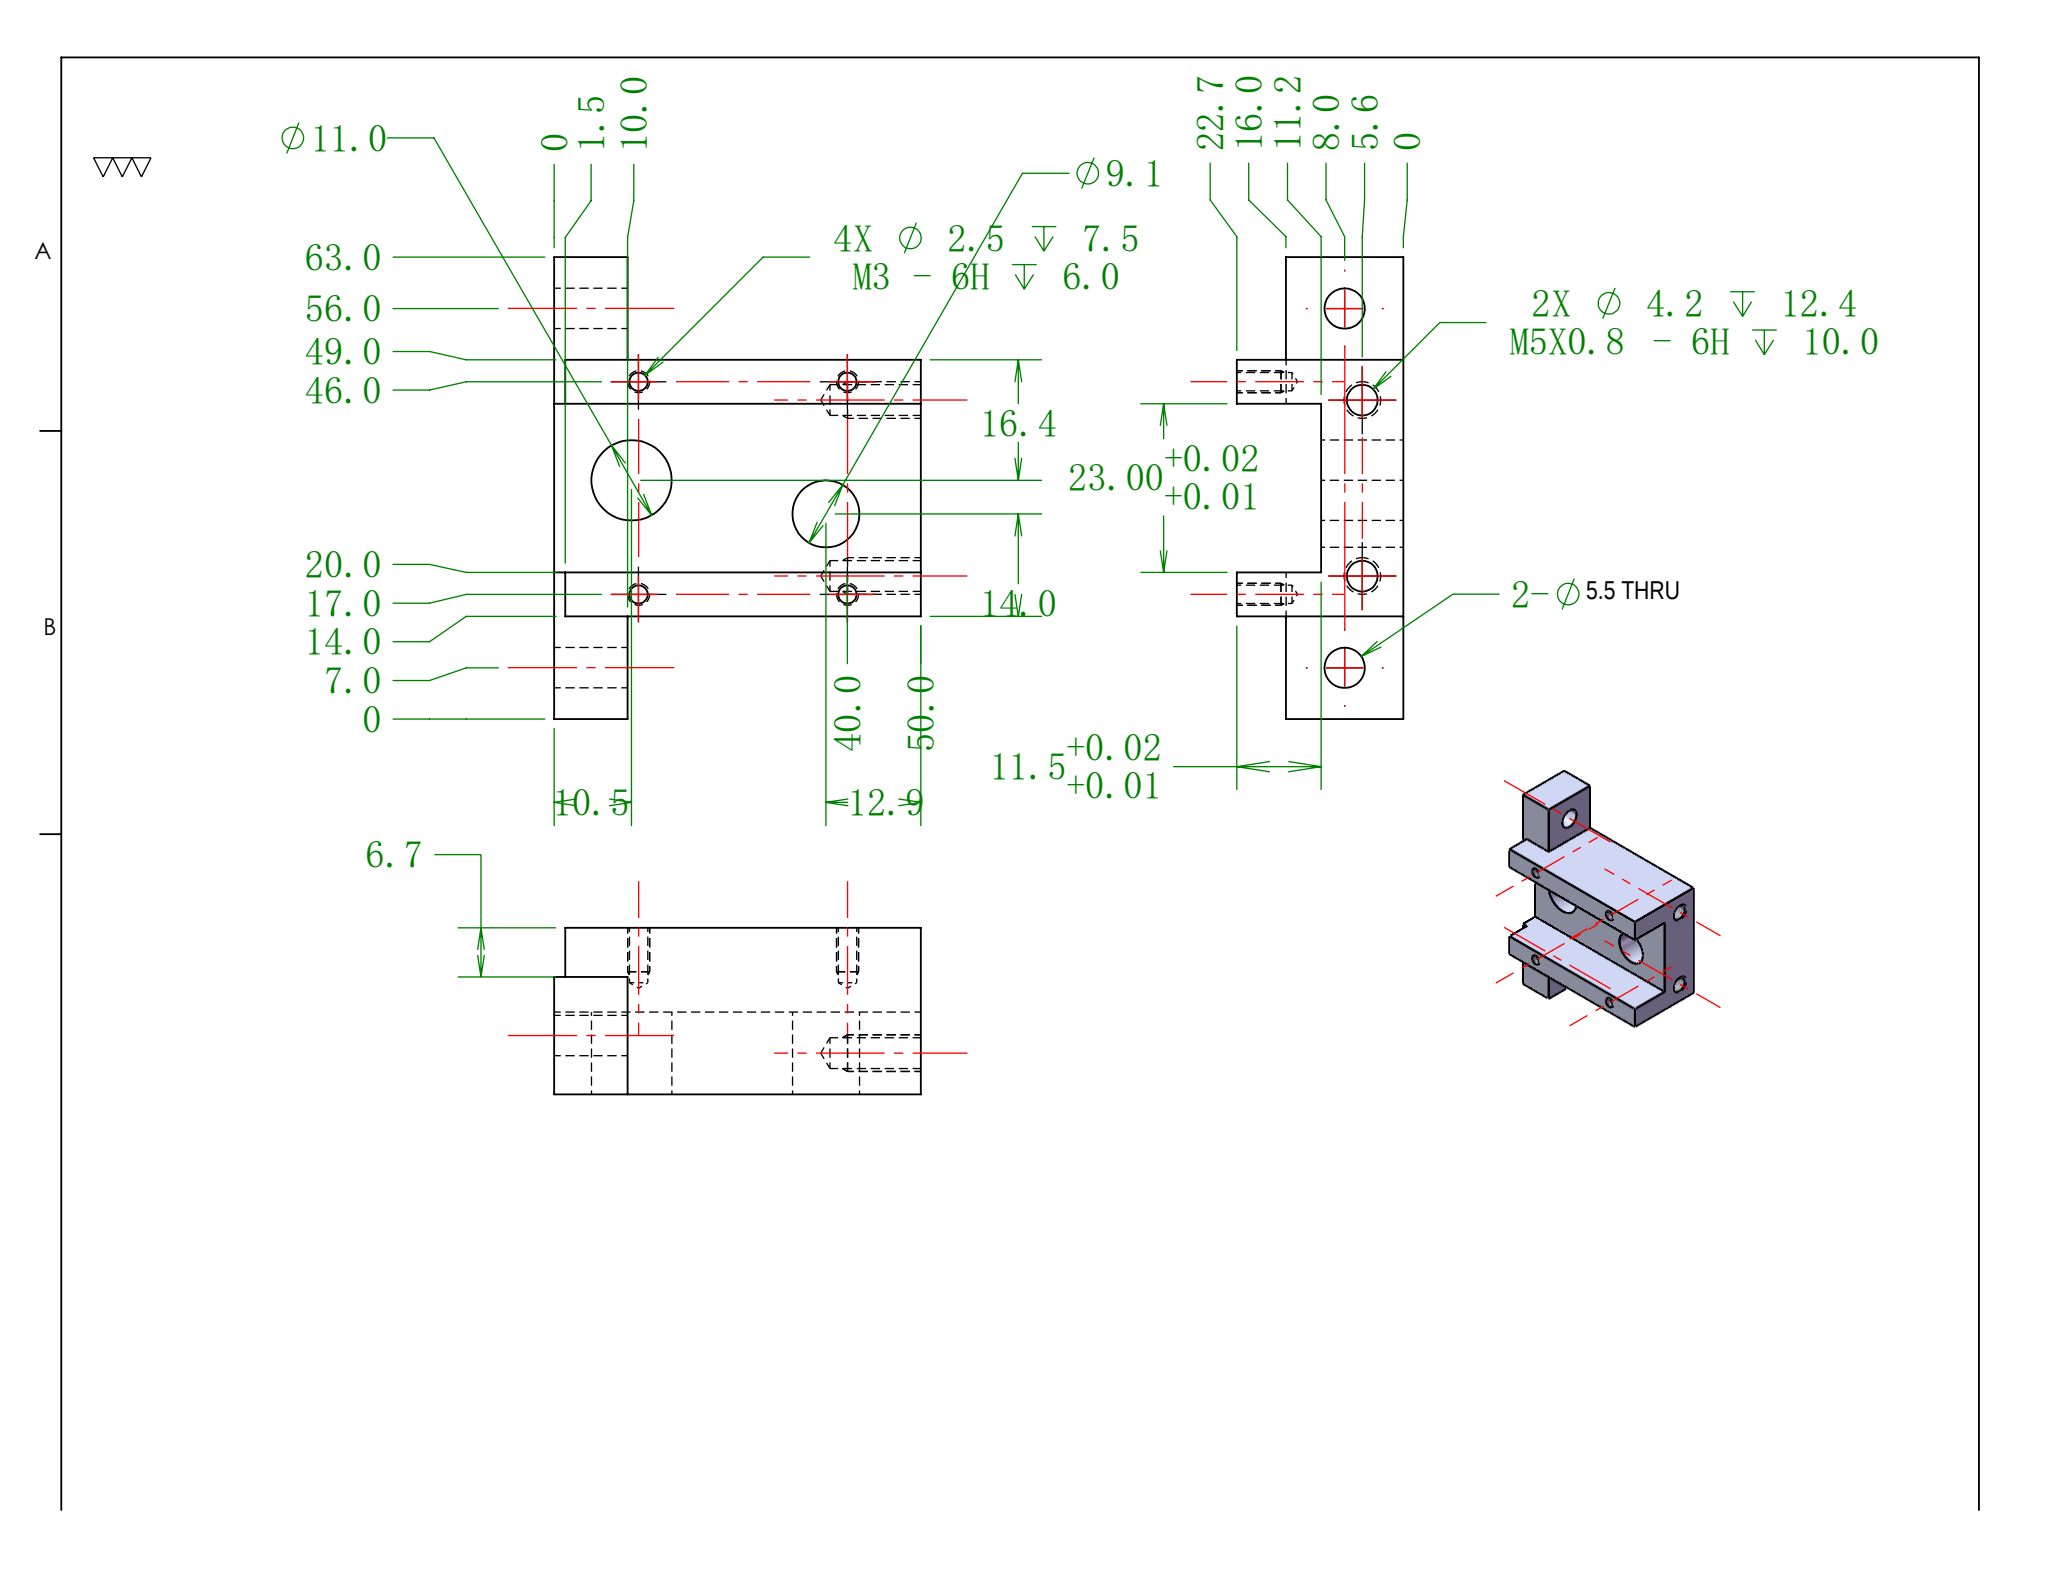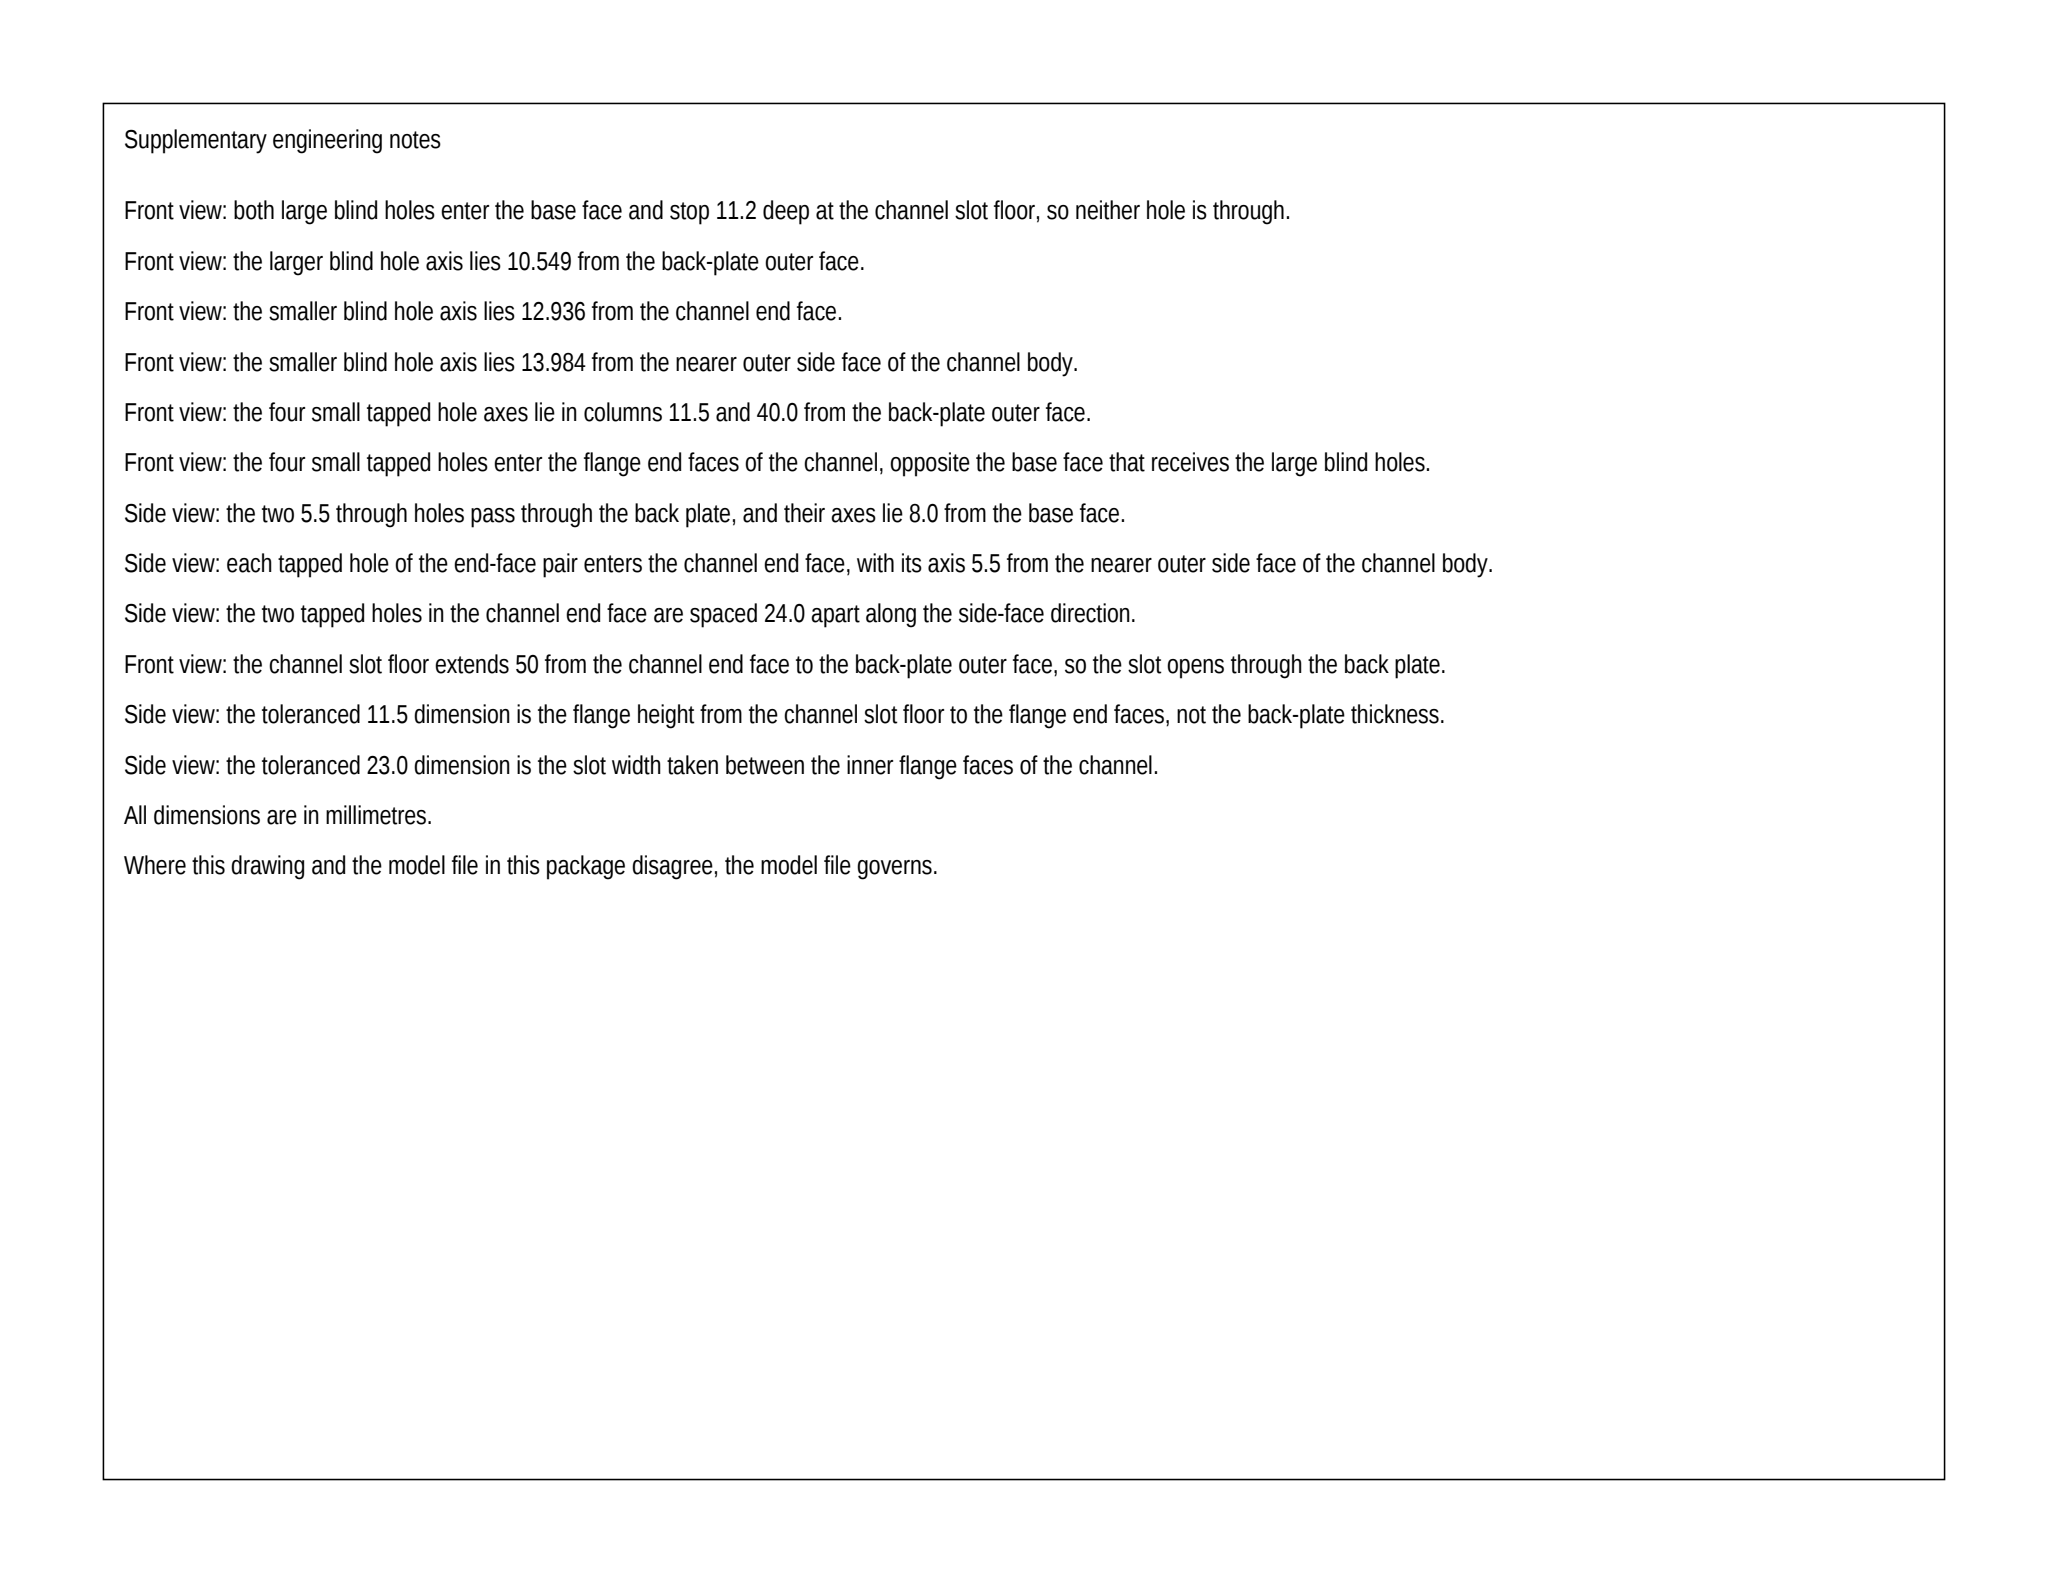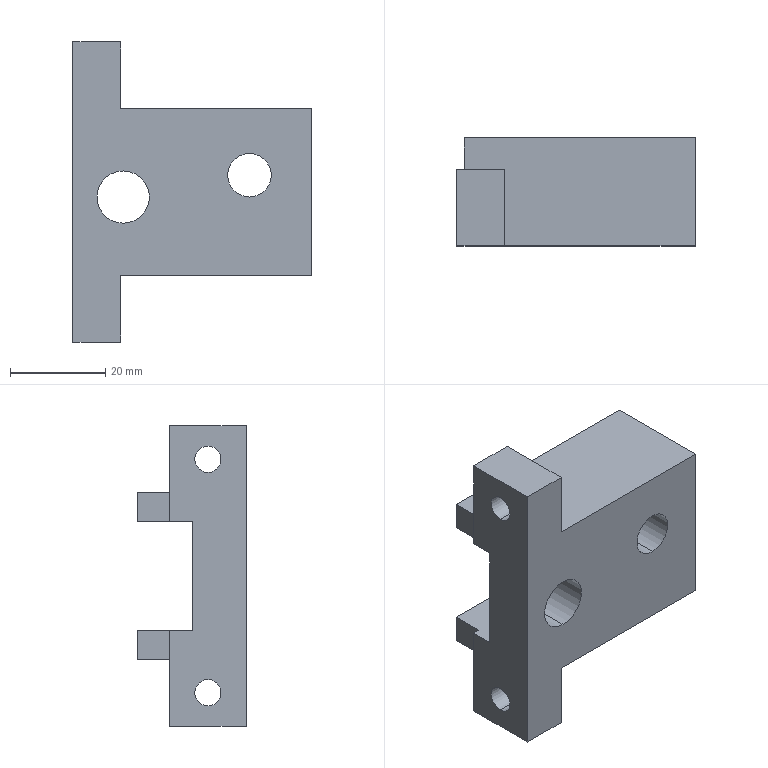Part | SolidWorks | mm | 1 solid | 50 faces | box 50 x 22.7 x 63 mm | volume 28084 mm3 | cylinder 20 | plane 18 | cone 12 | commonest cylinder face diameters 2.5 x8 4.2 x4 5.5 x4 10.967 x2 9.139 x2
Drawing notes:
2X M5X0.8 HOLE CL AT 19.5 & 43.5 FROM BTM FACE (0 DATUM) | from the solid: cylinders dia 4.2 axis x at z=19.5 and z=43.5, y=5.6; z=0 face is bbox min
FRONT VIEW: LH 4X M3 HOLE C/L AT 11.5 FROM 0 X-DATUM | from the solid: Ø2.5 y-axis cylinders at x=11.5, z=17.0 and z=46.0 (depth 7.5)
build123d program:
from build123d import *

# Parameters (mm, degrees)
SKETCH1_W                 = 35
SKETCH1_H                 = 22.7
EXTRUDE1_DEPTH            = 50
SKETCH2_W                 = 60
SKETCH2_H                 = 23
EXTRUDE2_DEPTH            = 11.5
SKETCH3_W                 = 10
SKETCH3_H                 = 14
EXTRUDE4_DEPTH            = 16
SKETCH6_R                 = 2.75
EXTRUDE5_DEPTH            = 68.203
M5X0_8_TAPPED_HOLE1_D     = 4.2
M5X0_8_TAPPED_HOLE1_DEPTH = 12.4
M5X0_8_TAPPED_HOLE1_TIP   = 1.262
M3_TAPPED_HOLE1_D         = 2.5
M3_TAPPED_HOLE1_DEPTH     = 7.5
M3_TAPPED_HOLE1_TIP       = 0.7511
SKETCH11_W                = 1.5
SKETCH11_H                = 6.7
EXTRUDE6_DEPTH            = 74.595
SKETCH12_R                = 5.484
SKETCH12_R_2              = 4.569
CUT_EXTRUDE1_DEPTH        = 31


with BuildPart() as part:
    # Sketch1 → Extrude1 (new body)
    with BuildSketch(Plane(origin=(0, 0, 0), x_dir=(0, 0, -1), z_dir=(1, 0, 0))):
        with Locations((17.5, 11.35)):
            Rectangle(SKETCH1_W, SKETCH1_H)
    extrude(amount=EXTRUDE1_DEPTH)

    # Sketch2 → Extrude2 (cut)
    with BuildSketch(Plane(origin=(0, 22.7, 0), x_dir=(1, 0, 0), z_dir=(0, 1, 0))):
        with Locations((30, 17.5)):
            Rectangle(SKETCH2_W, SKETCH2_H)
    extrude(amount=-EXTRUDE2_DEPTH, mode=Mode.SUBTRACT)

    # Sketch3 → Extrude4 (add)
    with BuildSketch(Plane.XZ):
        with Locations((5, 7)):
            Rectangle(SKETCH3_W, SKETCH3_H)
        with Locations((5, -42)):
            Rectangle(SKETCH3_W, SKETCH3_H)
    extrude(amount=-EXTRUDE4_DEPTH)

    # Sketch6 → Extrude5 (cut, through all)
    with BuildSketch(Plane(origin=(10, 0, 0), x_dir=(0, 0, -1), z_dir=(1, 0, 0))):
        with Locations((-7, 8)):
            Circle(SKETCH6_R)
        with Locations((42, 8)):
            Circle(SKETCH6_R)
    extrude(amount=-EXTRUDE5_DEPTH, mode=Mode.SUBTRACT)

    # M5x0.8 Tapped Hole1
    with Locations(Plane(origin=(50, 0, 0), x_dir=(0, 0, -1), z_dir=(1, 0, 0))):
        with Locations((29.5, 5.6), (5.5, 5.6)):
            Hole(M5X0_8_TAPPED_HOLE1_D / 2, depth=M5X0_8_TAPPED_HOLE1_DEPTH)
            with Locations((0, 0, -(M5X0_8_TAPPED_HOLE1_DEPTH + M5X0_8_TAPPED_HOLE1_TIP / 2))):  # 118° drill point
                Cone(0, M5X0_8_TAPPED_HOLE1_D / 2, M5X0_8_TAPPED_HOLE1_TIP, mode=Mode.SUBTRACT)

    # M3 Tapped Hole1
    with Locations(Plane(origin=(0, 22.7, 0), x_dir=(-1, 0, 0), z_dir=(0, 1, 0))):
        with Locations((-11.5, -32), (-40, -32), (-40, -3), (-11.5, -3)):
            Hole(M3_TAPPED_HOLE1_D / 2, depth=M3_TAPPED_HOLE1_DEPTH)
            with Locations((0, 0, -(M3_TAPPED_HOLE1_DEPTH + M3_TAPPED_HOLE1_TIP / 2))):  # 118° drill point
                Cone(0, M3_TAPPED_HOLE1_D / 2, M3_TAPPED_HOLE1_TIP, mode=Mode.SUBTRACT)

    # Sketch11 → Extrude6 (cut, through all)
    with BuildSketch(Plane(origin=(0, 0, -35), x_dir=(-1, 0, 0), z_dir=(0, 0, -1))):
        with Locations((-0.75, 19.35)):
            Rectangle(SKETCH11_W, SKETCH11_H)
    extrude(amount=-EXTRUDE6_DEPTH, mode=Mode.SUBTRACT)

    # Sketch12 → Cut-Extrude1 (cut)
    with BuildSketch(Plane(origin=(0, 11.2, 0), x_dir=(1, 0, 0), z_dir=(0, 1, 0))):
        with Locations(Location((10.549, 18.564, 0), (0, 0, 270))):
            Circle(SKETCH12_R)
        with Locations(Location((37.064, 13.984, 0), (0, 0, 270))):
            Circle(SKETCH12_R_2)
    extrude(amount=-CUT_EXTRUDE1_DEPTH, mode=Mode.SUBTRACT)


solid = part.part